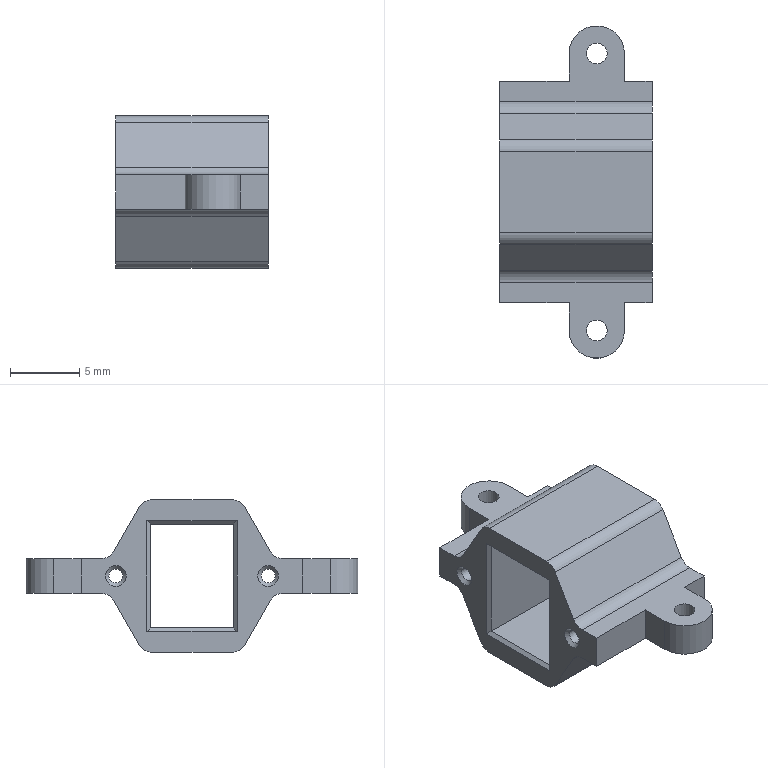Component | NX | DENGTOU | 1 solid | 48 faces | volume 864 mm3 | plane 30 | cylinder 16 | cone 2 | commonest cylinder face diameters 2 x8 4 x2 1.5 x2 2.5 x2 1 x2